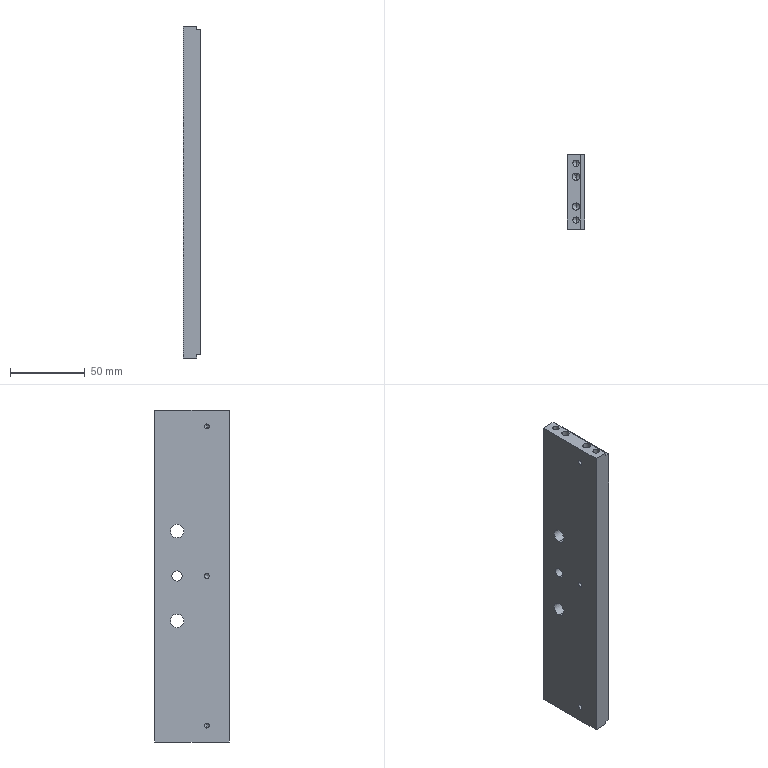Component | SolidWorks | 07-1111-1 | 1 solid | 64 faces | box 12 x 50 x 222 mm | volume 128732 mm3 | cylinder 32 | cone 22 | plane 10 | commonest cylinder face diameters 3.3 x10 5 x8 4.2 x8 9 x4 6.8 x2
build123d program:
from build123d import *

# Parameters (mm, degrees)
SKETCH5_W                           = 50
SKETCH5_H                           = 222
BOSS_EXTRUDE1_DEPTH                 = 12
M8_TAPPED_HOLE1_D                   = 6.8
M10X1_0_TAPPED_HOLE2_D              = 9
M5_TAPPED_HOLE1_AT_2_COUNT          = 2
M5_TAPPED_HOLE1_AT_2_PITCH          = 38
SIZE_MM_DOWEL_PIN_HOLE_1_AT_2_COUNT = 2
SIZE_MM_DOWEL_PIN_HOLE_1_AT_2_PITCH = 20
LPATTERN1_COUNT                     = 2
LPATTERN1_PITCH                     = 100
LPATTERN1_COL_COUNT                 = 2
LPATTERN1_COL_PITCH                 = 100
SKETCH1_W                           = 2.7
SKETCH1_H                           = 3.2
RELIEF_06_FLANGE_DEPTH              = 50


with BuildPart() as part:
    # Sketch5 → Boss-Extrude1 (new body)
    with BuildSketch(Plane(origin=(0, 0, 0), x_dir=(1, 0, 0), z_dir=(0, 1, 0))):
        Rectangle(SKETCH5_W, SKETCH5_H)
    extrude(amount=BOSS_EXTRUDE1_DEPTH)

    # M8 Tapped Hole1 (through all)
    with Locations(Plane(origin=(0, 0, 0), x_dir=(-1, 0, 0), z_dir=(0, -1, 0))):
        with Locations((-10, 0)):
            Hole(M8_TAPPED_HOLE1_D / 2)

    # M10x1.0 Tapped Hole2 (through all)
    with Locations(Plane(origin=(0, 0, 0), x_dir=(-1, 0, 0), z_dir=(0, -1, 0))):
        with Locations((-10, -30), (-10, 30)):
            Hole(M10X1_0_TAPPED_HOLE2_D / 2)

    # Sketch17 → M5 Tapped Hole1 (revolve, cut)
    with BuildSketch(Plane(origin=(-19, 6, 111), x_dir=(0, -1, 0), z_dir=(1, 0, 0))):
        Polygon((0, 0), (0, 13.662), (2.1, 12.4), (2.1, 0), align=None)
    m5_tapped_hole1 = revolve(axis=Axis((-19, 6, 117.35), (0, 0, -1)), mode=Mode.SUBTRACT)

    # M5 Tapped Hole1 at 2: M5 Tapped Hole1 ×2
    with Locations(*[(i * M5_TAPPED_HOLE1_AT_2_PITCH, 0, 0) for i in range(1, M5_TAPPED_HOLE1_AT_2_COUNT)]):
        add(m5_tapped_hole1, mode=Mode.SUBTRACT)

    # Sketch19 → Size mm Dowel Pin Hole 1 (revolve, cut)
    with BuildSketch(Plane(origin=(10, 6, 111), x_dir=(0, -1, 0), z_dir=(1, 0, 0))):
        Polygon((0, 0), (0, 13.902), (2.5, 12.4), (2.5, 0), align=None)
    size_mm_dowel_pin_hole_1 = revolve(axis=Axis((10, 6, 117.35), (0, 0, -1)), mode=Mode.SUBTRACT)

    # Size mm Dowel Pin Hole 1 at 2: Size mm Dowel Pin Hole 1 ×2
    with Locations(*[(-i * SIZE_MM_DOWEL_PIN_HOLE_1_AT_2_PITCH, 0, 0) for i in range(1, SIZE_MM_DOWEL_PIN_HOLE_1_AT_2_COUNT)]):
        add(size_mm_dowel_pin_hole_1, mode=Mode.SUBTRACT)

    # Mirror1: M5 Tapped Hole1, Size mm Dowel Pin Hole 1 across plane
    add(m5_tapped_hole1.mirror(Plane.XY), mode=Mode.SUBTRACT)
    add(size_mm_dowel_pin_hole_1.mirror(Plane.XY), mode=Mode.SUBTRACT)

    # Mirror1 copy 1 sketch → Mirror1 copy 1 (revolve, cut)
    with BuildSketch(Plane(origin=(19, 6, -111), x_dir=(0, -1, 0), z_dir=(1, 0, 0))):
        Polygon((0, 0), (0, -13.662), (2.1, -12.4), (2.1, 0), align=None)
    revolve(axis=Axis((19, 6, -117.35), (0, 0, -1)), mode=Mode.SUBTRACT)

    # Mirror1 copy 2 sketch → Mirror1 copy 2 (revolve, cut)
    with BuildSketch(Plane(origin=(-10, 6, -111), x_dir=(0, -1, 0), z_dir=(1, 0, 0))):
        Polygon((0, 0), (0, -13.902), (2.5, -12.4), (2.5, 0), align=None)
    revolve(axis=Axis((-10, 6, -117.35), (0, 0, -1)), mode=Mode.SUBTRACT)

    # Sketch21 → M4 Tapped Hole1 (revolve, cut)
    with BuildSketch(Plane(origin=(-10, 0, 0), x_dir=(0, 0, -1), z_dir=(1, 0, 0))):
        Polygon((0, 0), (0, 11.091), (1.65, 10.1), (1.65, 0), align=None)
    m4_tapped_hole1 = revolve(axis=Axis((-10, -6.35, 0), (0, 1, 0)), mode=Mode.SUBTRACT)

    # LPattern1: M4 Tapped Hole1 ×2
    with Locations(*[(0, 0, -i * LPATTERN1_PITCH) for i in range(1, LPATTERN1_COUNT)]):
        add(m4_tapped_hole1, mode=Mode.SUBTRACT)

    # LPattern1 col: M4 Tapped Hole1 ×2
    with Locations(*[(0, 0, i * LPATTERN1_COL_PITCH) for i in range(1, LPATTERN1_COL_COUNT)]):
        add(m4_tapped_hole1, mode=Mode.SUBTRACT)

    # Sketch1 → Relief-06-flange (cut, symmetric)
    with BuildSketch(Plane(origin=(0, 0, 0), x_dir=(0, 0, -1), z_dir=(1, 0, 0))):
        with Locations((-110.15, 10.9)):
            Rectangle(SKETCH1_W, SKETCH1_H)
        with Locations((110.15, 10.9)):
            Rectangle(SKETCH1_W, SKETCH1_H)
    extrude(amount=RELIEF_06_FLANGE_DEPTH, both=True, mode=Mode.SUBTRACT)


solid = part.part

# Placed as in the assembly
solid = solid.moved(Location((-165.072, 518.224, 1393.056), (180, 0, -90)))